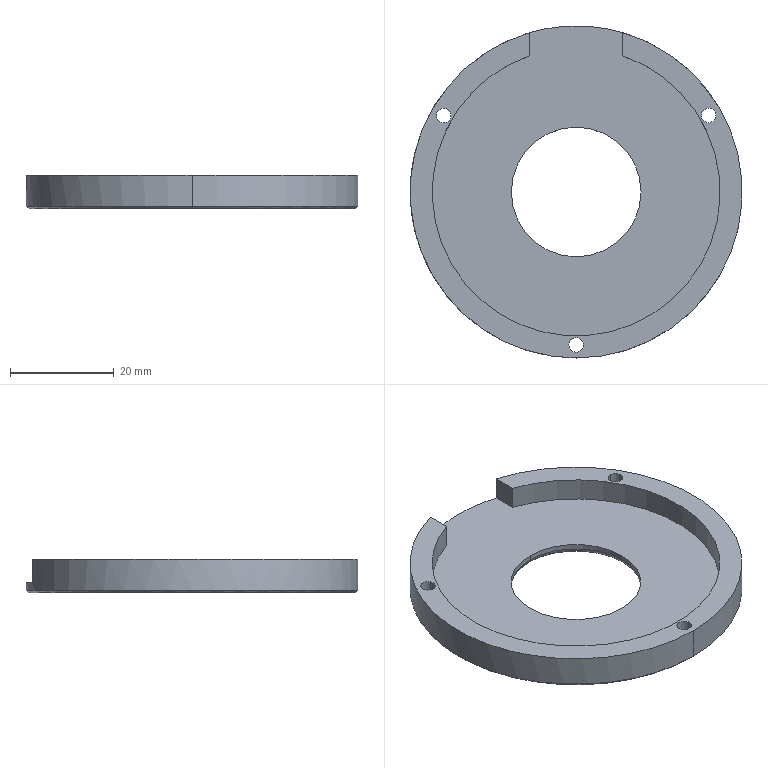CAM job | Mastercam | mm | 4 operations | part box 64 x 64 x 6.5
1. Contour (Ramp) | 10 - 10 平铣刀
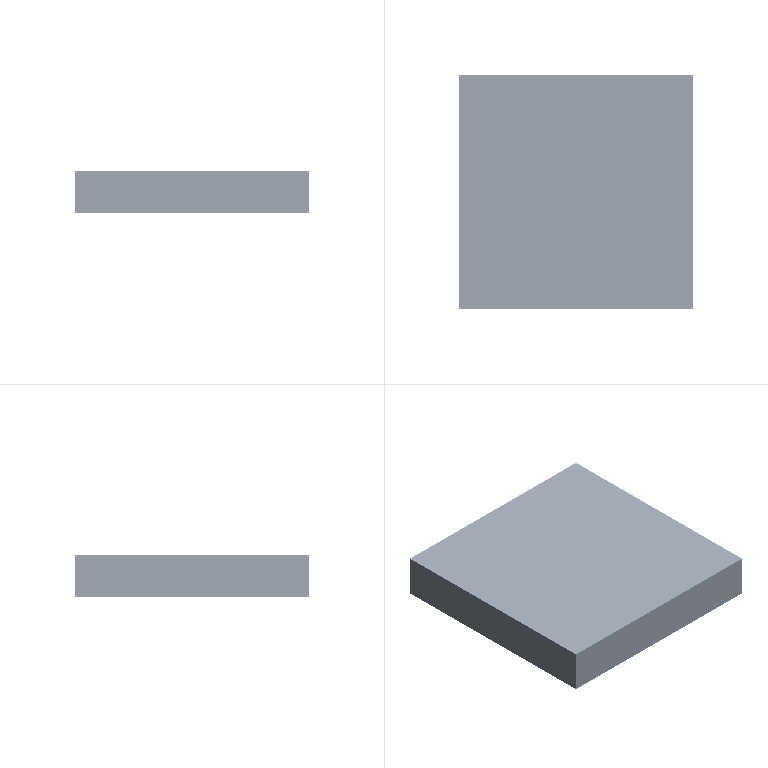2. Contour (2D) | 10 - 10 平铣刀
3. Drill/Counterbore | 7 - 4 倒角刀
4. Contour (2D chamfer) | 7 - 4 倒角刀